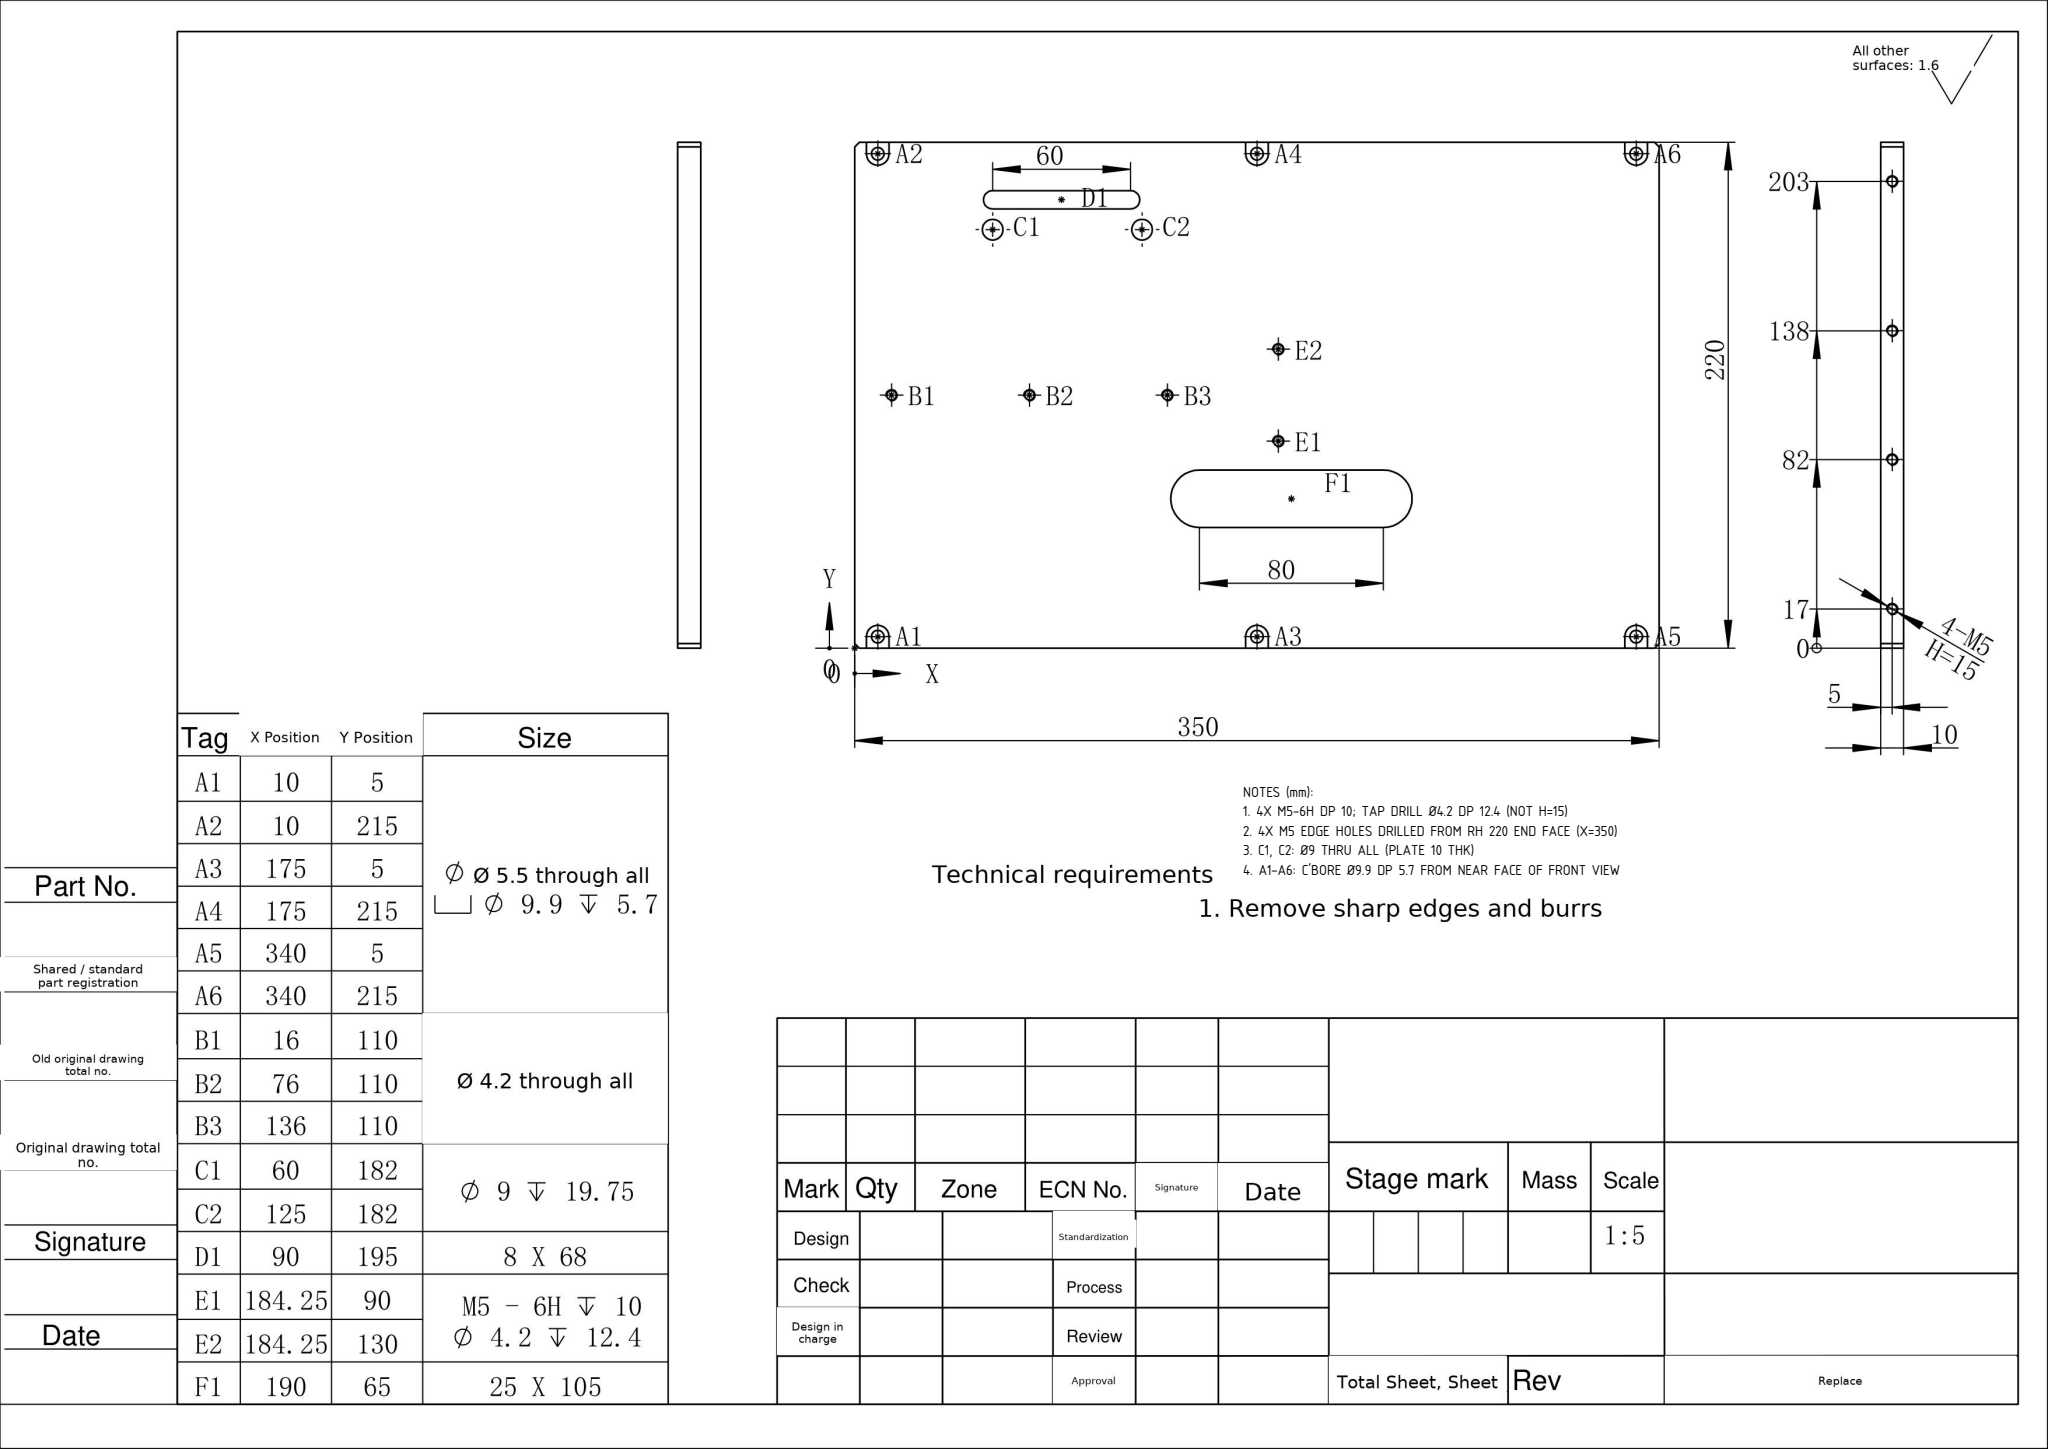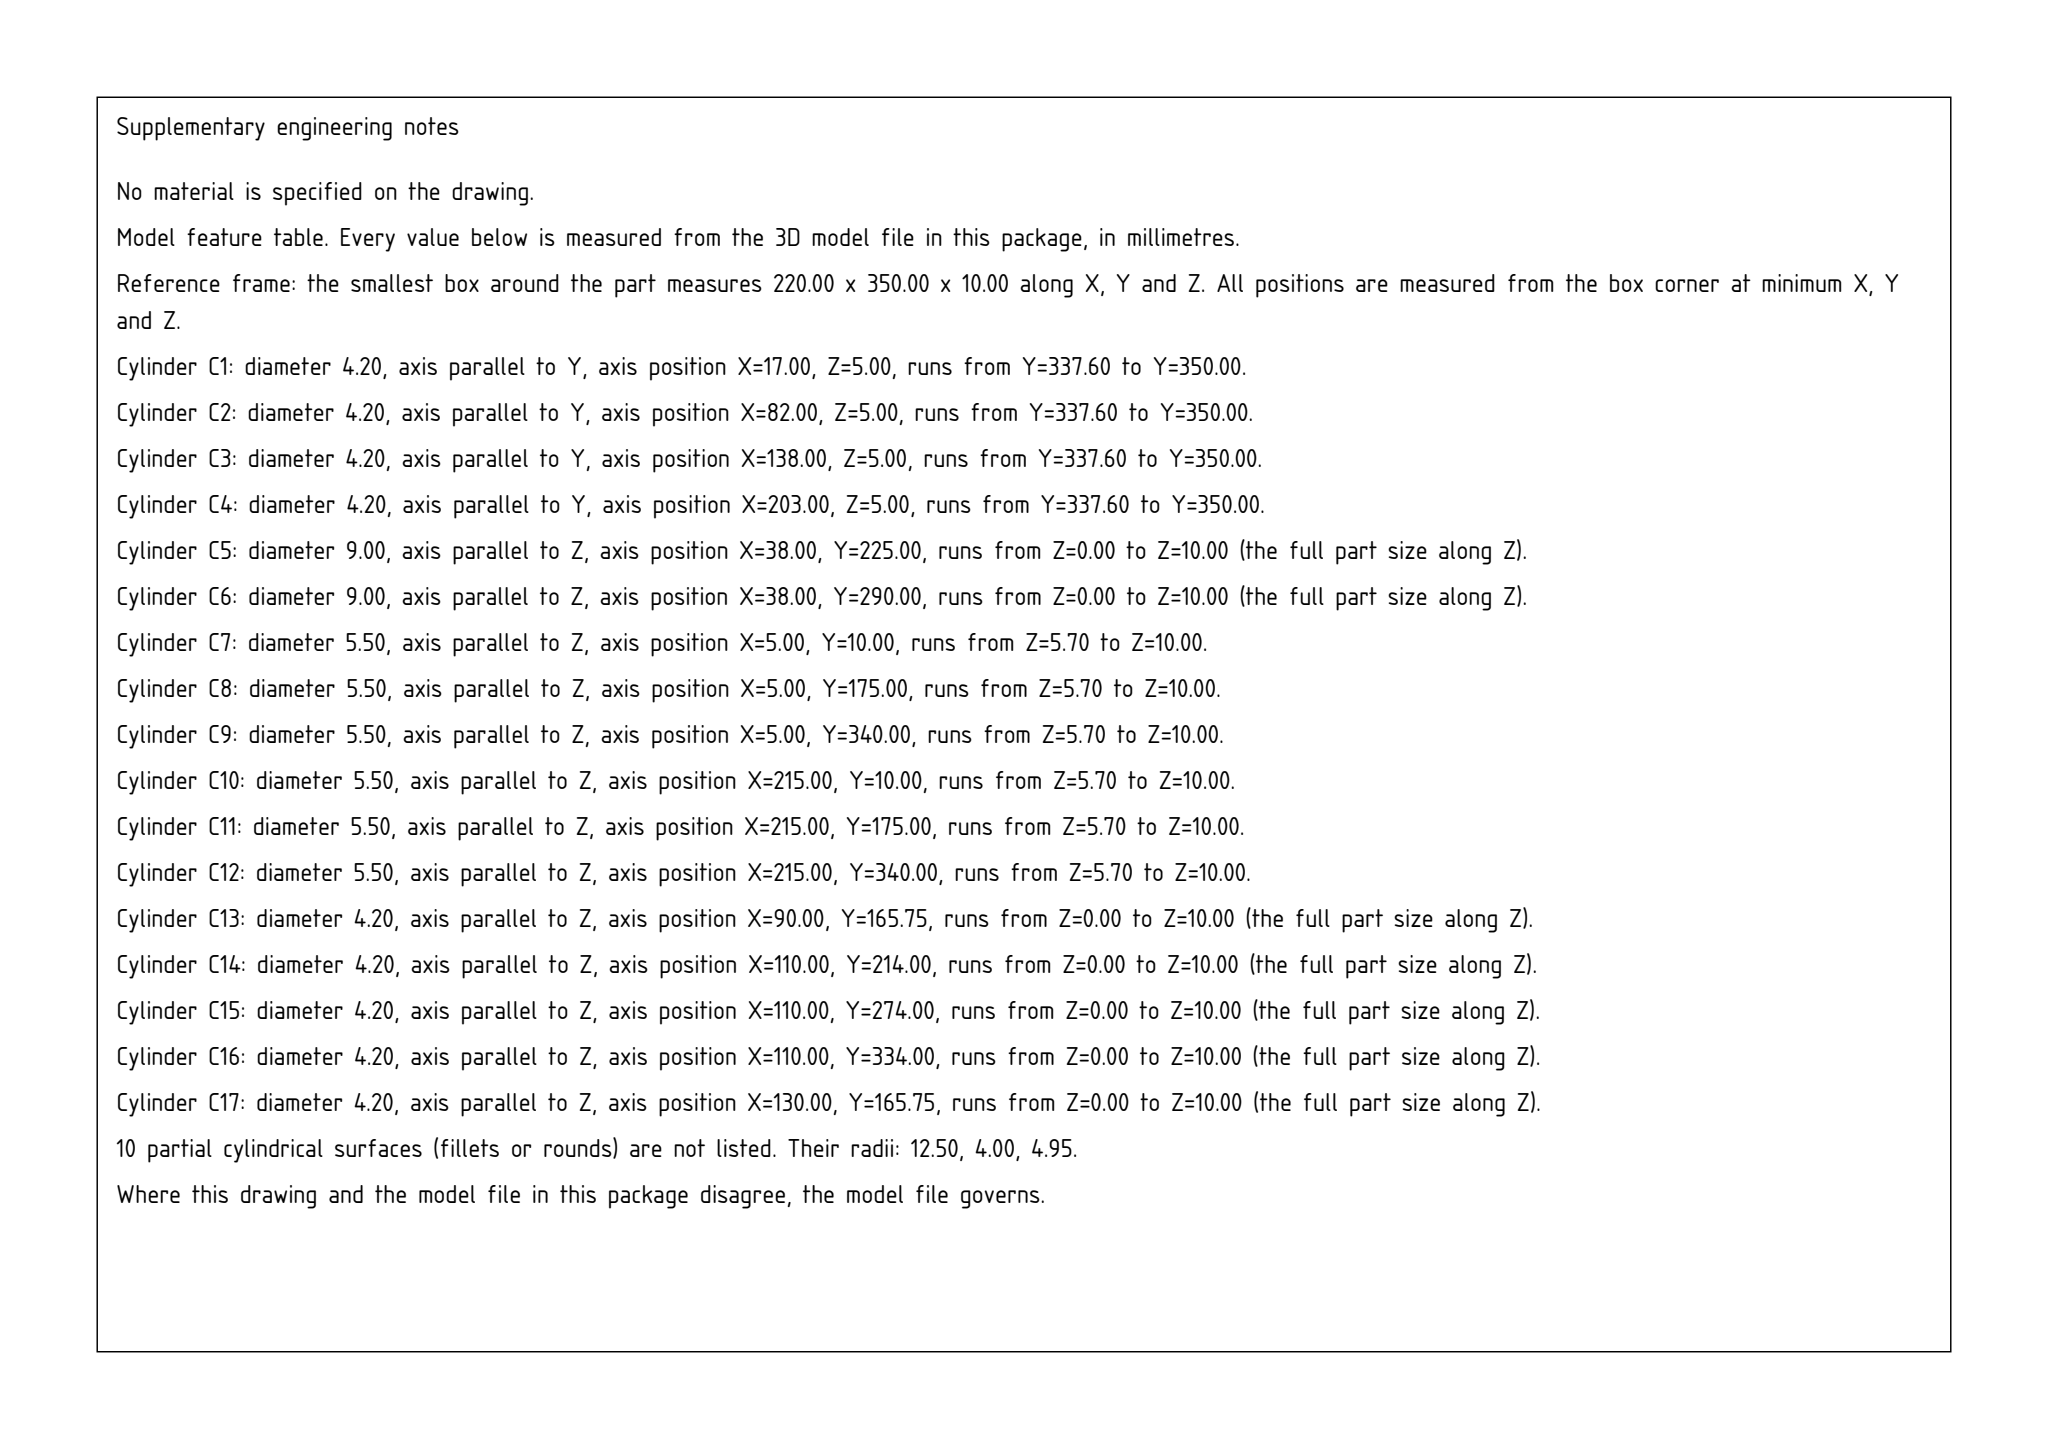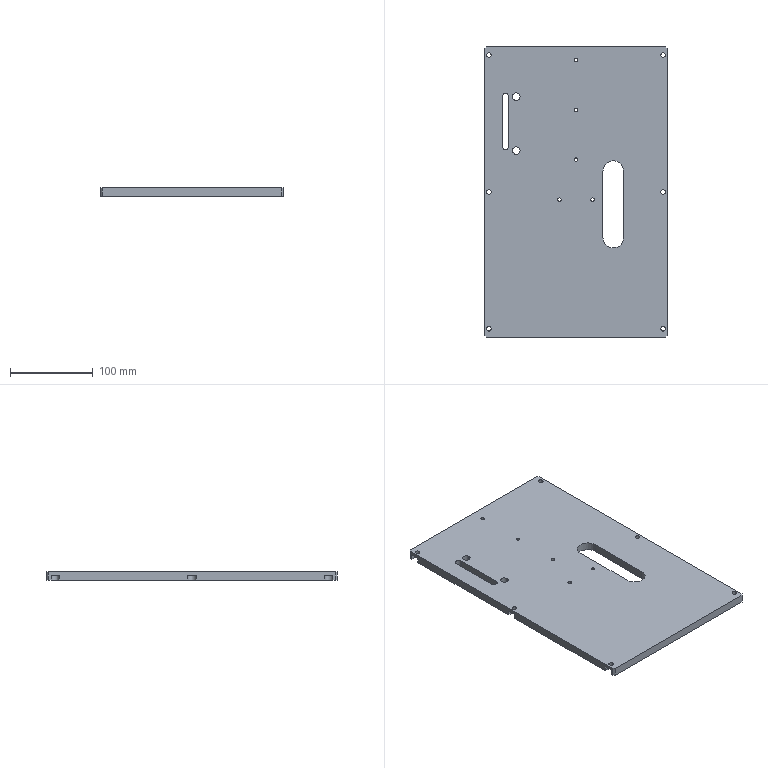Part | SolidWorks | mm | 1 solid | 87 faces | box 220 x 350 x 10 mm | volume 733411 mm3 | cylinder 47 | plane 32 | cone 8 | commonest cylinder face diameters 4.2 x18 5.5 x12 9.9 x9 9 x4 25 x2 8 x2
Drawing notes:
4X M5-6H DP 10; TAP DRILL Ø4.2 DP 12.4 (NOT H=15) | from the solid: Ø4.2 blind holes, axis y, len 12.4 at x=17/82/138/203, z=5; table E1 M5-6H ↧10 / Ø4.2 ↧12.4
4X M5 EDGE HOLES DRILLED FROM RH 220 END FACE (X=350) | from the solid: Ø4.2 y-axis holes start at y=0; drawing X = 350 - y, so entry at X=350 end face
C1, C2: Ø9 THRU ALL (PLATE 10 THK) | from the solid: Ø9 cylinders, axis z, length 10 = full 10 mm thickness at x=38, y=225/290
A1-A6: C'BORE Ø9.9 DP 5.7 FROM NEAR FACE OF FRONT VIEW | from the solid: Ø9.9 c'bores span z=0 to 5.7 (flat planes z=5.7), Ø5.5 len 4.3 to z=10; front view views z=0 face
build123d program:
from build123d import *

# Parameters (mm, degrees)
SKETCH1_W                                            = 220
SKETCH1_H                                            = 350
BOSS_EXTRUDE1_DEPTH                                  = 10
F_9_0_9_DIAMETER_HOLE1_D                             = 9
F_9_0_9_DIAMETER_HOLE1_DEPTH                         = 19.75
F_9_0_9_DIAMETER_HOLE1_TIP                           = 2.704
M5_TAPPED_HOLE1_D                                    = 4.2
M5_TAPPED_HOLE1_DEPTH                                = 12.4
M5_TAPPED_HOLE1_TIP                                  = 1.262
CHAMFER1_SIZE                                        = 2
HOLE_SIZE_ACCORDING_TO_HEXAGON_SOCKET_HE_D           = 5.5
HOLE_SIZE_ACCORDING_TO_HEXAGON_SOCKET_HE_CBORE_D     = 9.9
HOLE_SIZE_ACCORDING_TO_HEXAGON_SOCKET_HE_CBORE_DEPTH = 5.7
M5_TAPPED_HOLE2_D                                    = 4.2
M5_TAPPED_HOLE3_D                                    = 4.2
M5_TAPPED_HOLE3_DEPTH                                = 12.4
M5_TAPPED_HOLE3_TIP                                  = 1.262
CUT_EXTRUDE1_DEPTH                                   = 326.56
CUT_EXTRUDE2_DEPTH                                   = 326.56
SKETCH22_W                                           = 40.758
SKETCH22_H                                           = 9.9
CUT_EXTRUDE3_DEPTH                                   = 5.7


with BuildPart() as part:
    # Sketch1 → Boss-Extrude1 (new body)
    with BuildSketch(Plane.XY):
        with Locations((0, -131.25)):
            Rectangle(SKETCH1_W, SKETCH1_H)
    extrude(amount=BOSS_EXTRUDE1_DEPTH)

    # 9.0 _9_ Diameter Hole1
    with Locations(Plane(origin=(0, 0, 0), x_dir=(-1, 0, 0), z_dir=(0, 0, -1))):
        with Locations((72, -81.25), (72, -16.25)):
            Hole(F_9_0_9_DIAMETER_HOLE1_D / 2, depth=F_9_0_9_DIAMETER_HOLE1_DEPTH)
            with Locations((0, 0, -(F_9_0_9_DIAMETER_HOLE1_DEPTH + F_9_0_9_DIAMETER_HOLE1_TIP / 2))):  # 118° drill point
                Cone(0, F_9_0_9_DIAMETER_HOLE1_D / 2, F_9_0_9_DIAMETER_HOLE1_TIP, mode=Mode.SUBTRACT)

    # M5 Tapped Hole1
    with Locations(Plane(origin=(0, 0, 0), x_dir=(-1, 0, 0), z_dir=(0, 0, -1))):
        with Locations((20, -140.5), (-20, -140.5)):
            Hole(M5_TAPPED_HOLE1_D / 2, depth=M5_TAPPED_HOLE1_DEPTH)
            with Locations((0, 0, -(M5_TAPPED_HOLE1_DEPTH + M5_TAPPED_HOLE1_TIP / 2))):  # 118° drill point
                Cone(0, M5_TAPPED_HOLE1_D / 2, M5_TAPPED_HOLE1_TIP, mode=Mode.SUBTRACT)

    # Chamfer1
    chamfer1_edges = [part.edges().sort_by_distance(p)[0] for p in [
        (110, -306.25, 5),
        (-110, -306.25, 5),
        (-110, 43.75, 5),
        (110, 43.75, 5),
    ]]
    chamfer(chamfer1_edges, length=CHAMFER1_SIZE)

    # Hole Size_According to_Hexagon Socket He (through all)
    with Locations(Plane(origin=(0, 0, 0), x_dir=(-1, 0, 0), z_dir=(0, 0, -1))):
        with Locations((-105, -296.25), (-105, -131.25), (-105, 33.75), (105, -296.25), (105, -131.25), (105, 33.75)):
            CounterBoreHole(HOLE_SIZE_ACCORDING_TO_HEXAGON_SOCKET_HE_D / 2, HOLE_SIZE_ACCORDING_TO_HEXAGON_SOCKET_HE_CBORE_D / 2, HOLE_SIZE_ACCORDING_TO_HEXAGON_SOCKET_HE_CBORE_DEPTH)

    # M5 Tapped Hole2 (through all)
    with Locations(Plane(origin=(0, 0, 0), x_dir=(-1, 0, 0), z_dir=(0, 0, -1))):
        with Locations((0, -92.25), (0, -32.25), (0, 27.75)):
            Hole(M5_TAPPED_HOLE2_D / 2)

    # M5 Tapped Hole3
    with Locations(Plane(origin=(0, 43.75, 0), x_dir=(1, 0, 0), z_dir=(0, 1, 0))):
        with Locations((93, -5), (-93, -5), (-28, -5), (28, -5)):
            Hole(M5_TAPPED_HOLE3_D / 2, depth=M5_TAPPED_HOLE3_DEPTH)
            with Locations((0, 0, -(M5_TAPPED_HOLE3_DEPTH + M5_TAPPED_HOLE3_TIP / 2))):  # 118° drill point
                Cone(0, M5_TAPPED_HOLE3_D / 2, M5_TAPPED_HOLE3_TIP, mode=Mode.SUBTRACT)

    # Sketch20 → Cut-Extrude1 (cut, through all)
    with BuildSketch(Plane(origin=(0, 0, 0), x_dir=(-1, 0, 0), z_dir=(0, 0, -1))):
        with BuildLine():
            Line((-32.5, -106.25), (-32.5, -186.25))
            ThreePointArc((-32.5, -186.25), (-45, -198.75), (-57.5, -186.25))
            Line((-57.5, -186.25), (-57.5, -106.25))
            ThreePointArc((-57.5, -106.25), (-45, -93.75), (-32.5, -106.25))
        make_face()
    extrude(amount=-CUT_EXTRUDE1_DEPTH, mode=Mode.SUBTRACT)

    # Sketch21 → Cut-Extrude2 (cut, through all)
    with BuildSketch(Plane(origin=(0, 0, 0), x_dir=(-1, 0, 0), z_dir=(0, 0, -1))):
        with BuildLine():
            Line((89, -16.25), (89, -76.25))
            ThreePointArc((89, -76.25), (85, -80.25), (81, -76.25))
            Line((81, -76.25), (81, -16.25))
            ThreePointArc((81, -16.25), (85, -12.25), (89, -16.25))
        make_face()
    extrude(amount=-CUT_EXTRUDE2_DEPTH, mode=Mode.SUBTRACT)

    # Sketch22 → Cut-Extrude3 (cut)
    with BuildSketch(Plane(origin=(0, 0, 0), x_dir=(-1, 0, 0), z_dir=(0, 0, -1))):
        with Locations((-125.379, 33.75)):
            Rectangle(SKETCH22_W, SKETCH22_H)
        with Locations((-125.379, -131.25)):
            Rectangle(SKETCH22_W, SKETCH22_H)
        with Locations((-125.379, -296.25)):
            Rectangle(SKETCH22_W, SKETCH22_H)
        with Locations((125.379, -296.25)):
            Rectangle(SKETCH22_W, SKETCH22_H)
        with Locations((125.379, -131.25)):
            Rectangle(SKETCH22_W, SKETCH22_H)
        with Locations((125.379, 33.75)):
            Rectangle(SKETCH22_W, SKETCH22_H)
    extrude(amount=-CUT_EXTRUDE3_DEPTH, mode=Mode.SUBTRACT)


solid = part.part